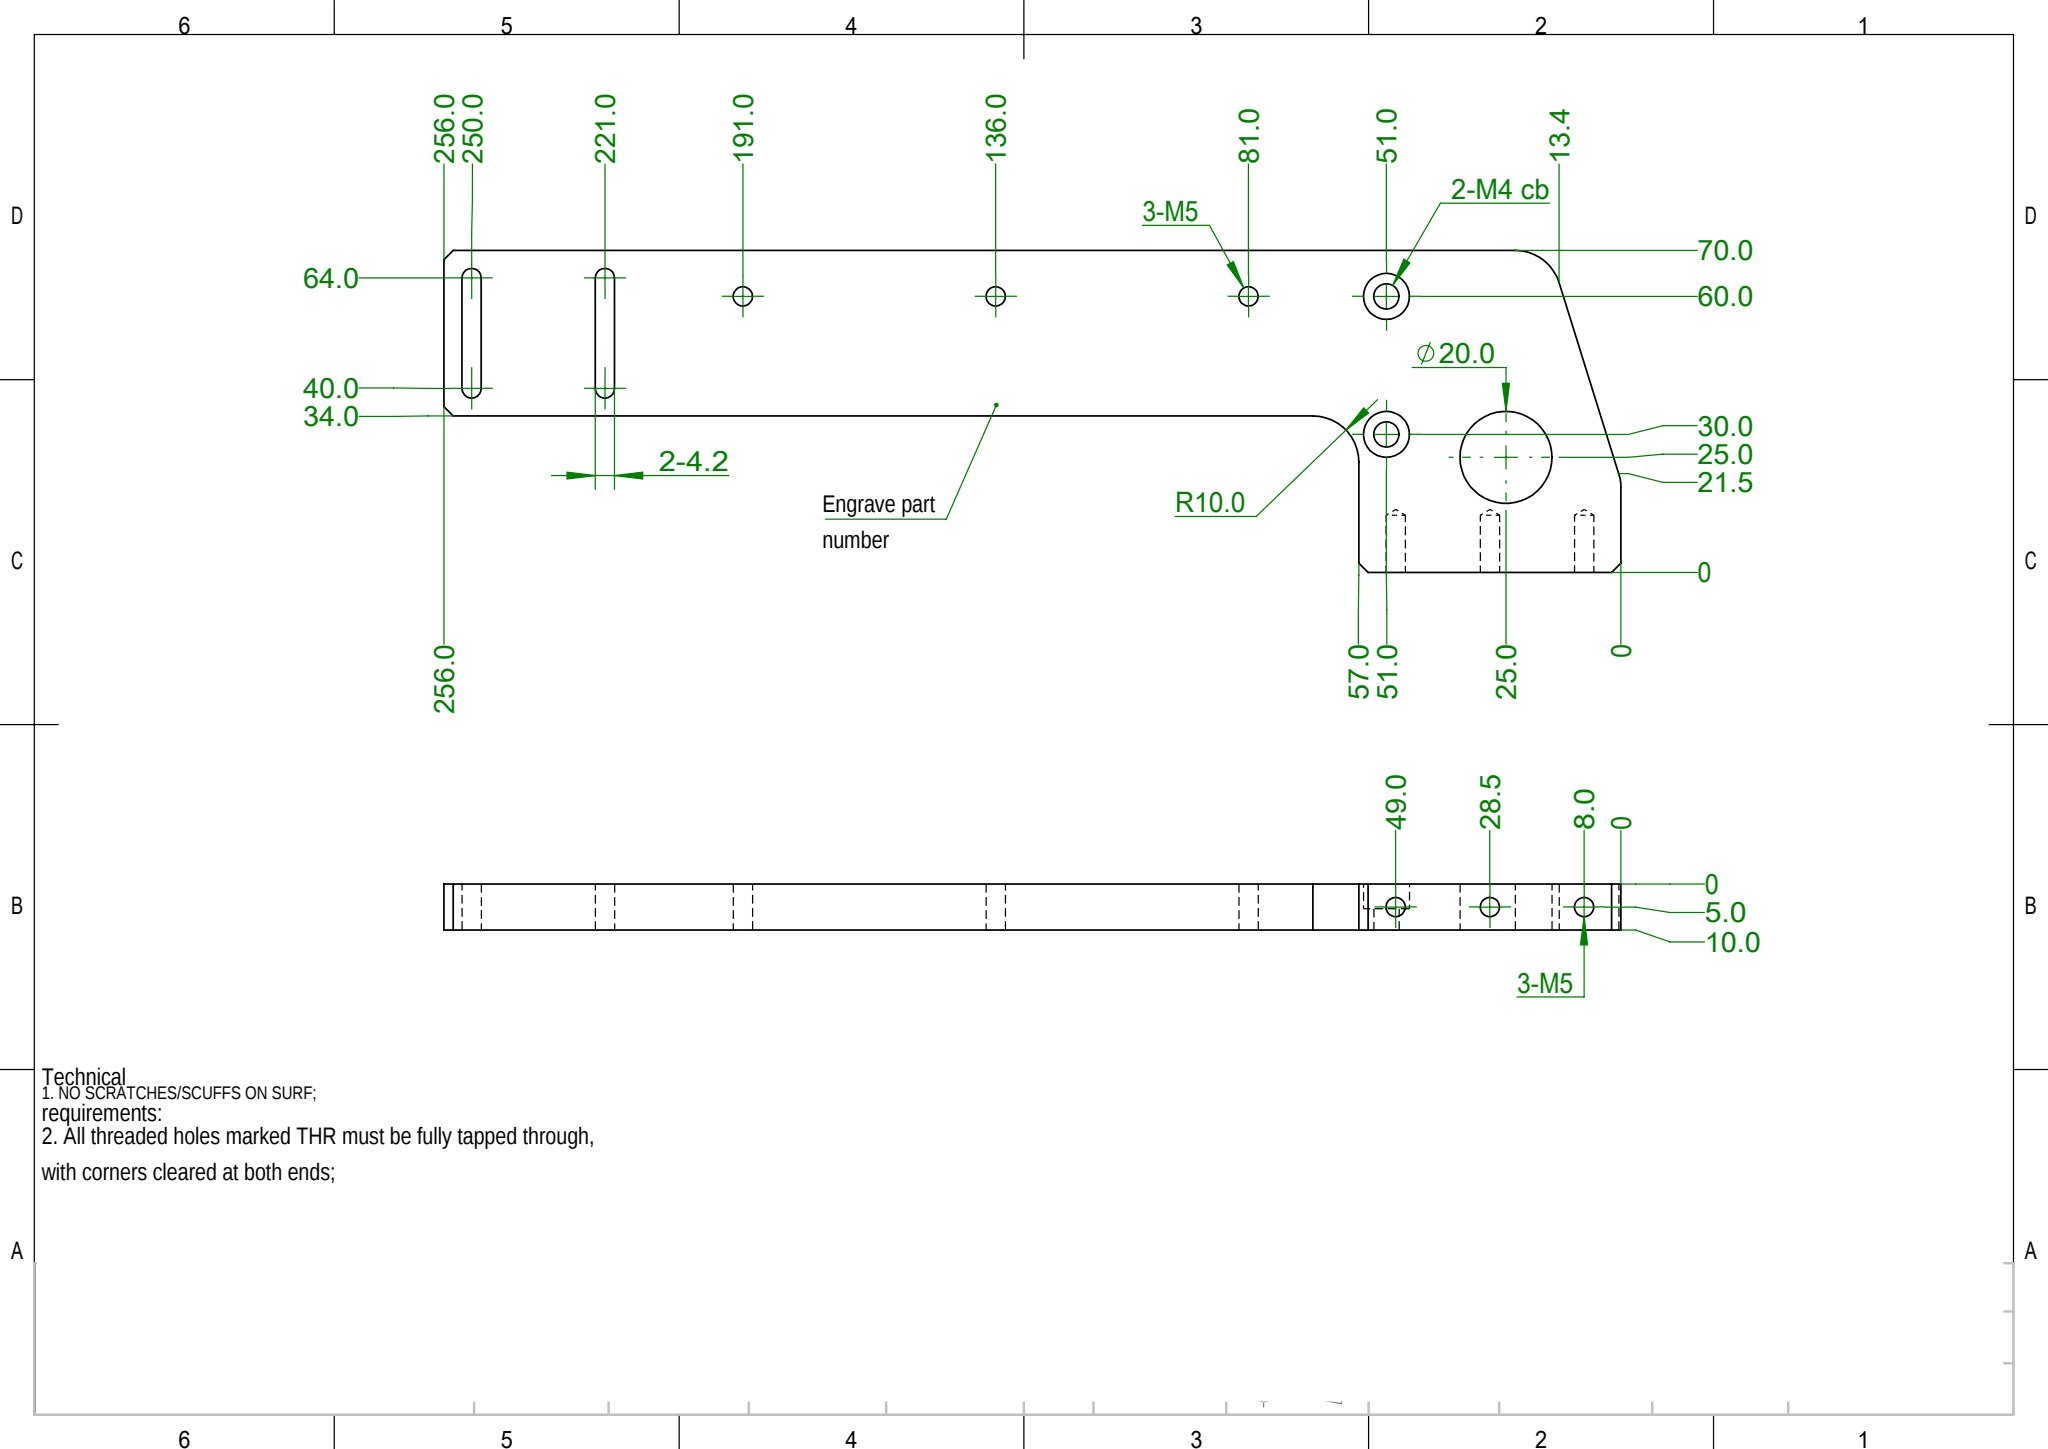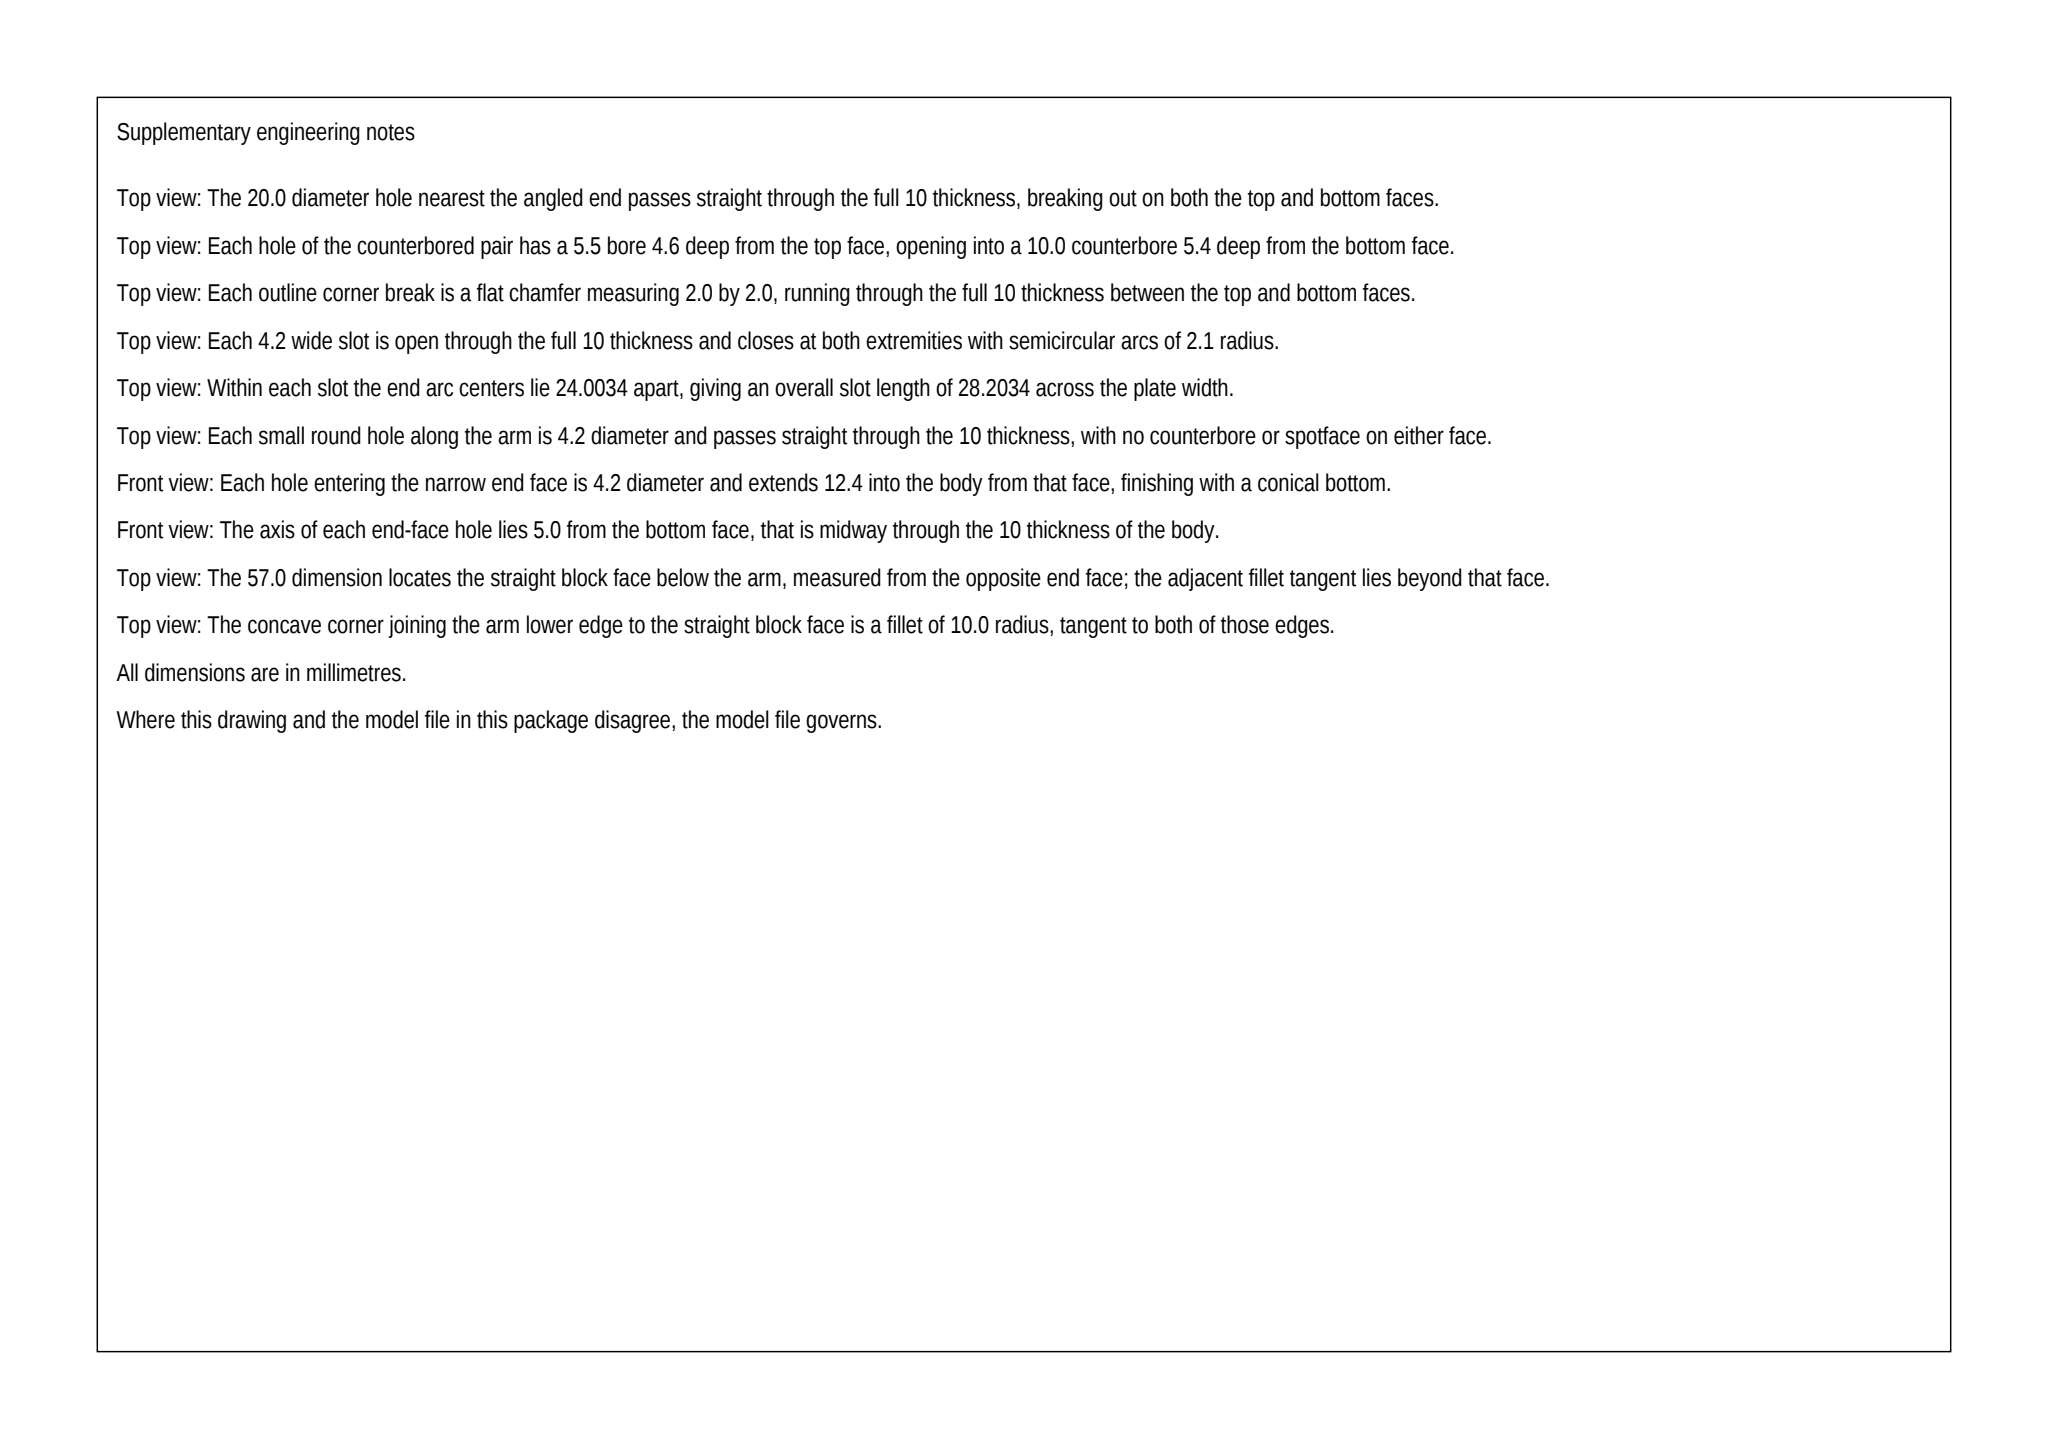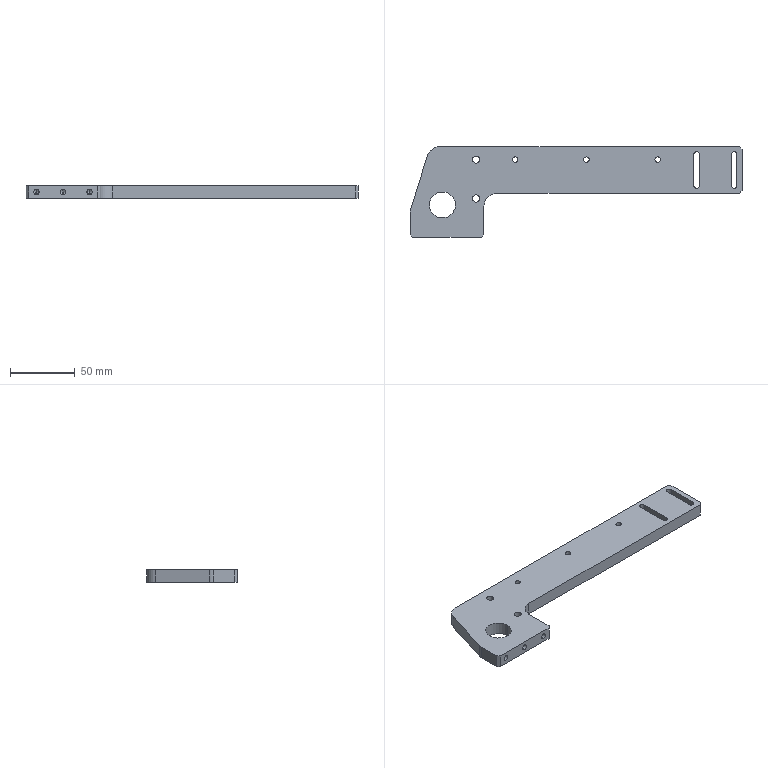Part | SolidWorks | mm | 1 solid | 54 faces | box 256 x 70 x 10 mm | volume 100217 mm3 | cylinder 29 | plane 19 | cone 6 | commonest cylinder face diameters 4.2 x16 20 x5 5.5 x4 10 x4
Drawing notes:
2-M4 CB: CBORE Ø10 DP 5.4 FROM TOP FACE, Ø5.5 THRU | from the solid: cyl Ø10 z-axis at (51,30)&(51,60) len 5.4 over Ø5.5 len 4.6 thru 10 thk
3-M5 IN Y0 FACE: Ø4.2 DRILL DP 12.4, THR PER NOTE 2 | from the solid: cyl Ø4.2 y-axis at x=8.0/28.5/49.0, z=5.0, length 12.4
SLANT EDGE ENDS: 2X R10, TAN TO 70.0 EDGE & 0 END FACE | from the solid: Ø20 z-cyl ctrs (10,18.47) tan x=0 and (22.98,60) tan y=70
ANGLED END EDGE: 17.35° FROM Y, TAN TO BOTH R10 ARCS | from the solid: line tangent to R10 ctrs (10,18.47)&(22.98,60): atan(12.98/41.53)=17.35°